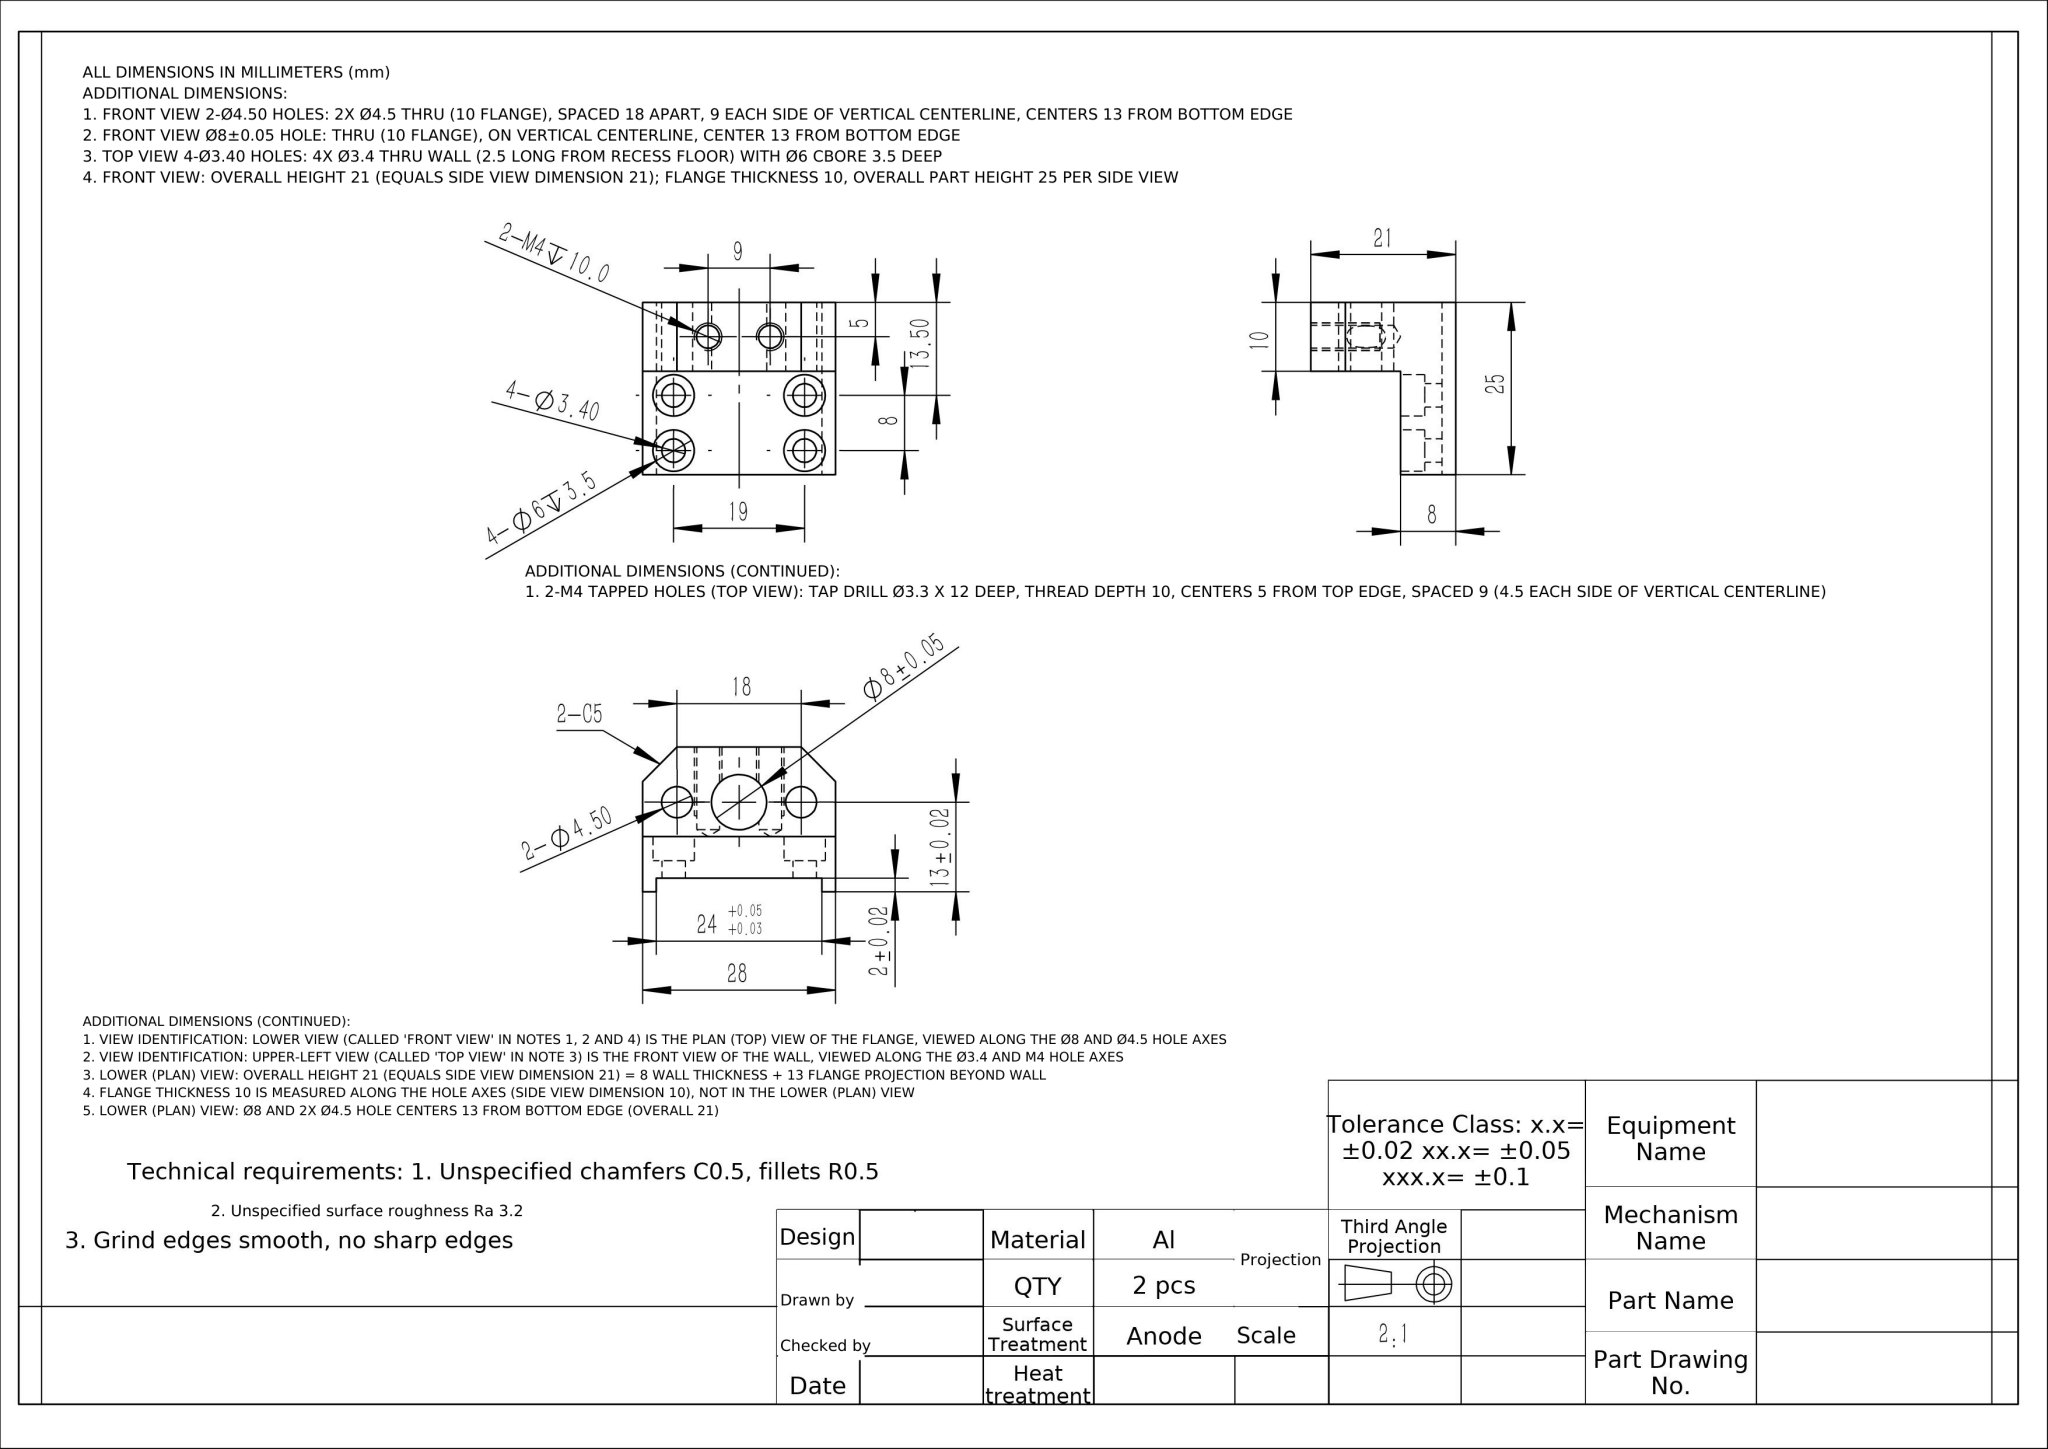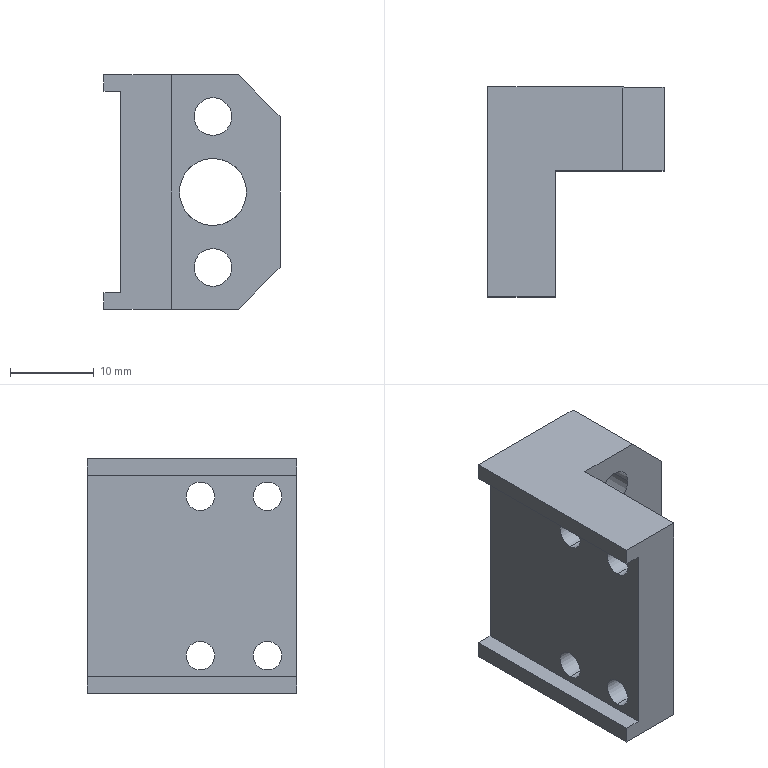Part | NX | mm | 1 solid | 48 faces | box 21 x 25 x 28 mm | volume 6290 mm3 | cylinder 26 | plane 18 | cone 4 | commonest cylinder face diameters 6 x8 3.4 x8 3.3 x4 4.5 x4 8 x2